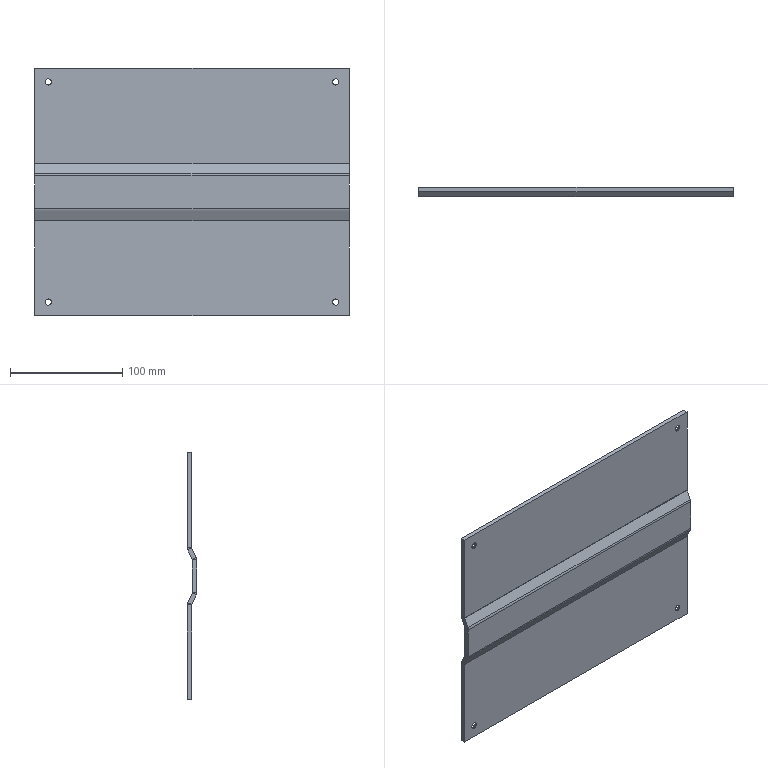Component | SolidWorks | Q1-A12-S21-Q4-01A-2 | 1 solid | 54 faces | volume 247766 mm3 | plane 30 | cylinder 16 | cone 8 | commonest cylinder face diameters 5.5 x8 9.473 x4 1.473 x4 | material SUS-304